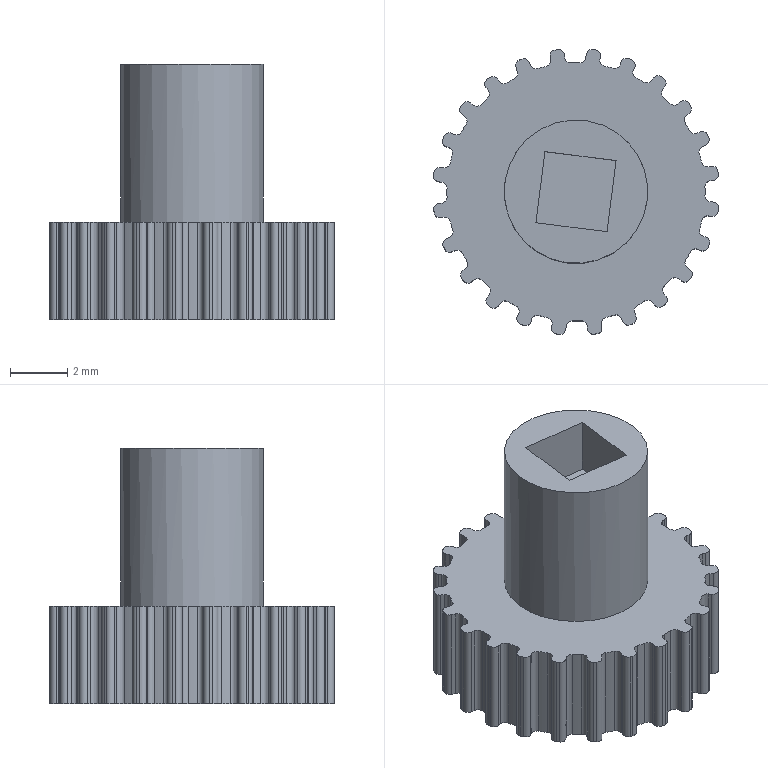Component | NX | INTERNAL_GEAR | 1 solid | 203 faces | volume 289 mm3 | cylinder 146 | plane 57 | commonest cylinder face diameters 0.4 x96 10 x24 9 x24 4 x1 5 x1